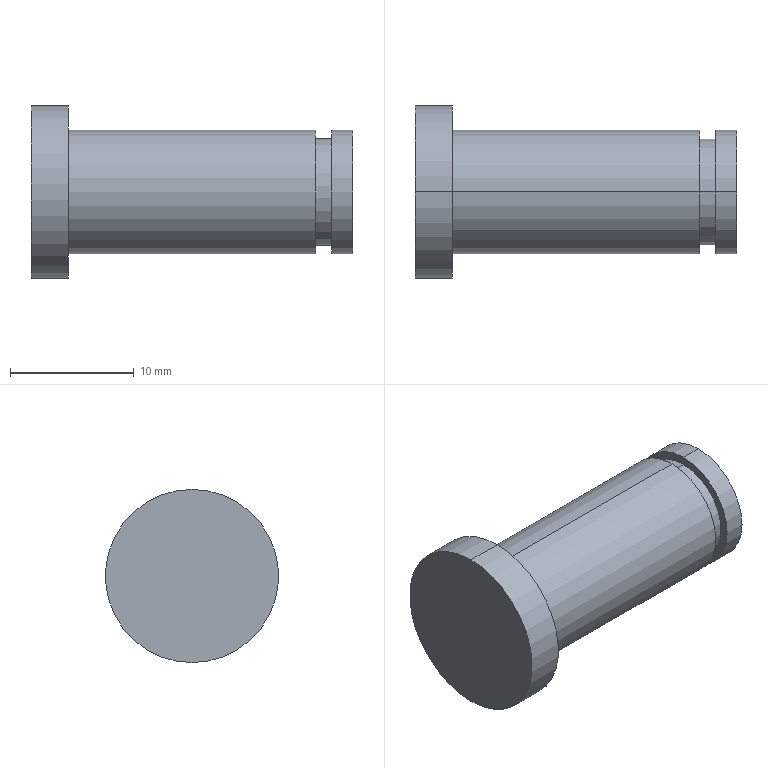Component | SolidWorks | OT-0200-012(PinShaft)-1 | 1 solid | 13 faces | box 26 x 14 x 14 mm | volume 2242 mm3 | cylinder 8 | plane 5 | commonest cylinder face diameters 10 x4 8.6 x2 14 x2 | material Plain Carbon Steel
build123d program:
from build123d import *


with BuildPart() as part:
    # Sketch1 → Revolve1 (revolve)
    with BuildSketch(Plane(origin=(0, 0, 0), x_dir=(1, 0, 0), z_dir=(0, 1, 0))):
        Polygon((0, 7), (0, 0), (26, 0), (26, 5), (24.3, 5), (24.3, 4.3), (23, 4.3), (23, 5), (3, 5), (3, 7), align=None)
    revolve(axis=Axis((26, 0, 0), (-1, 0, 0)))


solid = part.part

# Placed as in the assembly
solid = solid.moved(Location((187, 104.973, -26.996), (0, 0, 0)))
STEP:
#1=CARTESIAN_POINT('',(8.319,4.133,-1.26));
#2=VERTEX_POINT('',#1);
#3=CARTESIAN_POINT('',(8.319,4.133,-0.866));
#4=VERTEX_POINT('',#3);
#5=CARTESIAN_POINT('',(8.319,4.133,-1.063));
#6=DIRECTION('',(1.,0.,0.));
#7=DIRECTION('',(0.,0.,-1.));
#8=AXIS2_PLACEMENT_3D('',#5,#6,#7);
#9=CIRCLE('',#8,0.1969);
#10=EDGE_CURVE('',#2,#4,#9,.T.);
#11=ORIENTED_EDGE('',*,*,#10,.T.);
#12=CARTESIAN_POINT('',(8.386,4.133,-0.866));
#13=VERTEX_POINT('',#12);
#14=CARTESIAN_POINT('',(8.386,4.133,-0.866));
#15=DIRECTION('',(1.,0.,0.));
#16=VECTOR('',#15,39.37);
#17=LINE('',#14,#16);
#18=EDGE_CURVE('',#4,#13,#17,.T.);
#19=ORIENTED_EDGE('',*,*,#18,.T.);
#20=CARTESIAN_POINT('',(8.386,4.133,-1.26));
#21=VERTEX_POINT('',#20);
#22=CARTESIAN_POINT('',(8.386,4.133,-1.063));
#23=DIRECTION('',(1.,0.,0.));
#24=DIRECTION('',(0.,0.,-1.));
#25=AXIS2_PLACEMENT_3D('',#22,#23,#24);
#26=CIRCLE('',#25,0.1969);
#27=EDGE_CURVE('',#21,#13,#26,.T.);
#28=ORIENTED_EDGE('',*,*,#27,.F.);
#29=CARTESIAN_POINT('',(8.386,4.133,-1.26));
#30=DIRECTION('',(1.,0.,0.));
#31=VECTOR('',#30,39.37);
#32=LINE('',#29,#31);
#33=EDGE_CURVE('',#2,#21,#32,.T.);
#34=ORIENTED_EDGE('',*,*,#33,.F.);
#35=EDGE_LOOP('',(#11,#19,#28,#34));
#36=FACE_OUTER_BOUND('',#35,.T.);
#37=CARTESIAN_POINT('',(8.386,4.133,-1.063));
#38=DIRECTION('',(1.,0.,0.));
#39=DIRECTION('',(0.,0.,-1.));
#40=AXIS2_PLACEMENT_3D('',#37,#38,#39);
#41=CYLINDRICAL_SURFACE('',#40,0.1969);
#42=ADVANCED_FACE('',(#36),#41,.T.);
#43=CARTESIAN_POINT('',(8.268,4.133,-1.232));
#44=VERTEX_POINT('',#43);
#45=CARTESIAN_POINT('',(8.268,4.133,-0.8935));
#46=VERTEX_POINT('',#45);
#47=CARTESIAN_POINT('',(8.268,4.133,-1.063));
#48=DIRECTION('',(1.,0.,0.));
#49=DIRECTION('',(0.,0.,-1.));
#50=AXIS2_PLACEMENT_3D('',#47,#48,#49);
#51=CIRCLE('',#50,0.1693);
#52=EDGE_CURVE('',#44,#46,#51,.T.);
#53=ORIENTED_EDGE('',*,*,#52,.T.);
#54=CARTESIAN_POINT('',(8.319,4.133,-0.8935));
#55=VERTEX_POINT('',#54);
#56=CARTESIAN_POINT('',(8.386,4.133,-0.8935));
#57=DIRECTION('',(1.,0.,0.));
#58=VECTOR('',#57,39.37);
#59=LINE('',#56,#58);
#60=EDGE_CURVE('',#46,#55,#59,.T.);
#61=ORIENTED_EDGE('',*,*,#60,.T.);
#62=CARTESIAN_POINT('',(8.319,4.133,-1.232));
#63=VERTEX_POINT('',#62);
#64=CARTESIAN_POINT('',(8.319,4.133,-1.063));
#65=DIRECTION('',(1.,0.,0.));
#66=DIRECTION('',(0.,0.,-1.));
#67=AXIS2_PLACEMENT_3D('',#64,#65,#66);
#68=CIRCLE('',#67,0.1693);
#69=EDGE_CURVE('',#63,#55,#68,.T.);
#70=ORIENTED_EDGE('',*,*,#69,.F.);
#71=CARTESIAN_POINT('',(8.386,4.133,-1.232));
#72=DIRECTION('',(1.,0.,0.));
#73=VECTOR('',#72,39.37);
#74=LINE('',#71,#73);
#75=EDGE_CURVE('',#44,#63,#74,.T.);
#76=ORIENTED_EDGE('',*,*,#75,.F.);
#77=EDGE_LOOP('',(#53,#61,#70,#76));
#78=FACE_OUTER_BOUND('',#77,.T.);
#79=CARTESIAN_POINT('',(8.386,4.133,-1.063));
#80=DIRECTION('',(1.,0.,0.));
#81=DIRECTION('',(0.,0.,-1.));
#82=AXIS2_PLACEMENT_3D('',#79,#80,#81);
#83=CYLINDRICAL_SURFACE('',#82,0.1693);
#84=ADVANCED_FACE('',(#78),#83,.T.);
#85=CARTESIAN_POINT('',(7.48,4.133,-1.26));
#86=VERTEX_POINT('',#85);
#87=CARTESIAN_POINT('',(7.48,4.133,-0.866));
#88=VERTEX_POINT('',#87);
#89=CARTESIAN_POINT('',(7.48,4.133,-1.063));
#90=DIRECTION('',(1.,0.,0.));
#91=DIRECTION('',(0.,0.,-1.));
#92=AXIS2_PLACEMENT_3D('',#89,#90,#91);
#93=CIRCLE('',#92,0.1969);
#94=EDGE_CURVE('',#86,#88,#93,.T.);
#95=ORIENTED_EDGE('',*,*,#94,.T.);
#96=CARTESIAN_POINT('',(8.268,4.133,-0.866));
#97=VERTEX_POINT('',#96);
#98=CARTESIAN_POINT('',(8.386,4.133,-0.866));
#99=DIRECTION('',(1.,0.,0.));
#100=VECTOR('',#99,39.37);
#101=LINE('',#98,#100);
#102=EDGE_CURVE('',#88,#97,#101,.T.);
#103=ORIENTED_EDGE('',*,*,#102,.T.);
#104=CARTESIAN_POINT('',(8.268,4.133,-1.26));
#105=VERTEX_POINT('',#104);
#106=CARTESIAN_POINT('',(8.268,4.133,-1.063));
#107=DIRECTION('',(1.,0.,0.));
#108=DIRECTION('',(0.,0.,-1.));
#109=AXIS2_PLACEMENT_3D('',#106,#107,#108);
#110=CIRCLE('',#109,0.1969);
#111=EDGE_CURVE('',#105,#97,#110,.T.);
#112=ORIENTED_EDGE('',*,*,#111,.F.);
#113=CARTESIAN_POINT('',(8.386,4.133,-1.26));
#114=DIRECTION('',(1.,0.,0.));
#115=VECTOR('',#114,39.37);
#116=LINE('',#113,#115);
#117=EDGE_CURVE('',#86,#105,#116,.T.);
#118=ORIENTED_EDGE('',*,*,#117,.F.);
#119=EDGE_LOOP('',(#95,#103,#112,#118));
#120=FACE_OUTER_BOUND('',#119,.T.);
#121=CARTESIAN_POINT('',(8.386,4.133,-1.063));
#122=DIRECTION('',(1.,0.,0.));
#123=DIRECTION('',(0.,0.,-1.));
#124=AXIS2_PLACEMENT_3D('',#121,#122,#123);
#125=CYLINDRICAL_SURFACE('',#124,0.1969);
#126=ADVANCED_FACE('',(#120),#125,.T.);
#127=CARTESIAN_POINT('',(7.362,4.133,-1.338));
#128=VERTEX_POINT('',#127);
#129=CARTESIAN_POINT('',(7.362,4.133,-0.7872));
#130=VERTEX_POINT('',#129);
#131=CARTESIAN_POINT('',(7.362,4.133,-1.063));
#132=DIRECTION('',(1.,0.,0.));
#133=DIRECTION('',(0.,0.,-1.));
#134=AXIS2_PLACEMENT_3D('',#131,#132,#133);
#135=CIRCLE('',#134,0.2756);
#136=EDGE_CURVE('',#128,#130,#135,.T.);
#137=ORIENTED_EDGE('',*,*,#136,.T.);
#138=CARTESIAN_POINT('',(7.48,4.133,-0.7872));
#139=VERTEX_POINT('',#138);
#140=CARTESIAN_POINT('',(8.386,4.133,-0.7872));
#141=DIRECTION('',(1.,0.,0.));
#142=VECTOR('',#141,39.37);
#143=LINE('',#140,#142);
#144=EDGE_CURVE('',#130,#139,#143,.T.);
#145=ORIENTED_EDGE('',*,*,#144,.T.);
#146=CARTESIAN_POINT('',(7.48,4.133,-1.338));
#147=VERTEX_POINT('',#146);
#148=CARTESIAN_POINT('',(7.48,4.133,-1.063));
#149=DIRECTION('',(1.,0.,0.));
#150=DIRECTION('',(0.,0.,-1.));
#151=AXIS2_PLACEMENT_3D('',#148,#149,#150);
#152=CIRCLE('',#151,0.2756);
#153=EDGE_CURVE('',#147,#139,#152,.T.);
#154=ORIENTED_EDGE('',*,*,#153,.F.);
#155=CARTESIAN_POINT('',(8.386,4.133,-1.338));
#156=DIRECTION('',(1.,0.,0.));
#157=VECTOR('',#156,39.37);
#158=LINE('',#155,#157);
#159=EDGE_CURVE('',#128,#147,#158,.T.);
#160=ORIENTED_EDGE('',*,*,#159,.F.);
#161=EDGE_LOOP('',(#137,#145,#154,#160));
#162=FACE_OUTER_BOUND('',#161,.T.);
#163=CARTESIAN_POINT('',(8.386,4.133,-1.063));
#164=DIRECTION('',(1.,0.,0.));
#165=DIRECTION('',(0.,0.,-1.));
#166=AXIS2_PLACEMENT_3D('',#163,#164,#165);
#167=CYLINDRICAL_SURFACE('',#166,0.2756);
#168=ADVANCED_FACE('',(#162),#167,.T.);
#169=ORIENTED_EDGE('',*,*,#144,.F.);
#170=CARTESIAN_POINT('',(7.362,4.133,-1.063));
#171=DIRECTION('',(1.,0.,0.));
#172=DIRECTION('',(0.,0.,-1.));
#173=AXIS2_PLACEMENT_3D('',#170,#171,#172);
#174=CIRCLE('',#173,0.2756);
#175=EDGE_CURVE('',#130,#128,#174,.T.);
#176=ORIENTED_EDGE('',*,*,#175,.T.);
#177=ORIENTED_EDGE('',*,*,#159,.T.);
#178=CARTESIAN_POINT('',(7.48,4.133,-1.063));
#179=DIRECTION('',(1.,0.,0.));
#180=DIRECTION('',(0.,0.,-1.));
#181=AXIS2_PLACEMENT_3D('',#178,#179,#180);
#182=CIRCLE('',#181,0.2756);
#183=EDGE_CURVE('',#139,#147,#182,.T.);
#184=ORIENTED_EDGE('',*,*,#183,.F.);
#185=EDGE_LOOP('',(#169,#176,#177,#184));
#186=FACE_OUTER_BOUND('',#185,.T.);
#187=CARTESIAN_POINT('',(8.386,4.133,-1.063));
#188=DIRECTION('',(1.,0.,0.));
#189=DIRECTION('',(0.,0.,-1.));
#190=AXIS2_PLACEMENT_3D('',#187,#188,#189);
#191=CYLINDRICAL_SURFACE('',#190,0.2756);
#192=ADVANCED_FACE('',(#186),#191,.T.);
#193=ORIENTED_EDGE('',*,*,#153,.T.);
#194=ORIENTED_EDGE('',*,*,#183,.T.);
#195=EDGE_LOOP('',(#193,#194));
#196=FACE_OUTER_BOUND('',#195,.T.);
#197=ORIENTED_EDGE('',*,*,#94,.F.);
#198=CARTESIAN_POINT('',(7.48,4.133,-1.063));
#199=DIRECTION('',(1.,0.,0.));
#200=DIRECTION('',(0.,0.,-1.));
#201=AXIS2_PLACEMENT_3D('',#198,#199,#200);
#202=CIRCLE('',#201,0.1969);
#203=EDGE_CURVE('',#88,#86,#202,.T.);
#204=ORIENTED_EDGE('',*,*,#203,.F.);
#205=EDGE_LOOP('',(#197,#204));
#206=FACE_BOUND('',#205,.T.);
#207=CARTESIAN_POINT('',(7.48,4.133,-1.338));
#208=DIRECTION('',(1.,0.,0.));
#209=DIRECTION('',(0.,0.,-1.));
#210=AXIS2_PLACEMENT_3D('',#207,#208,#209);
#211=PLANE('',#210);
#212=ADVANCED_FACE('',(#196,#206),#211,.T.);
#213=ORIENTED_EDGE('',*,*,#102,.F.);
#214=ORIENTED_EDGE('',*,*,#203,.T.);
#215=ORIENTED_EDGE('',*,*,#117,.T.);
#216=CARTESIAN_POINT('',(8.268,4.133,-1.063));
#217=DIRECTION('',(1.,0.,0.));
#218=DIRECTION('',(0.,0.,-1.));
#219=AXIS2_PLACEMENT_3D('',#216,#217,#218);
#220=CIRCLE('',#219,0.1969);
#221=EDGE_CURVE('',#97,#105,#220,.T.);
#222=ORIENTED_EDGE('',*,*,#221,.F.);
#223=EDGE_LOOP('',(#213,#214,#215,#222));
#224=FACE_OUTER_BOUND('',#223,.T.);
#225=CARTESIAN_POINT('',(8.386,4.133,-1.063));
#226=DIRECTION('',(1.,0.,0.));
#227=DIRECTION('',(0.,0.,-1.));
#228=AXIS2_PLACEMENT_3D('',#225,#226,#227);
#229=CYLINDRICAL_SURFACE('',#228,0.1969);
#230=ADVANCED_FACE('',(#224),#229,.T.);
#231=ORIENTED_EDGE('',*,*,#111,.T.);
#232=ORIENTED_EDGE('',*,*,#221,.T.);
#233=EDGE_LOOP('',(#231,#232));
#234=FACE_OUTER_BOUND('',#233,.T.);
#235=ORIENTED_EDGE('',*,*,#52,.F.);
#236=CARTESIAN_POINT('',(8.268,4.133,-1.063));
#237=DIRECTION('',(1.,0.,0.));
#238=DIRECTION('',(0.,0.,-1.));
#239=AXIS2_PLACEMENT_3D('',#236,#237,#238);
#240=CIRCLE('',#239,0.1693);
#241=EDGE_CURVE('',#46,#44,#240,.T.);
#242=ORIENTED_EDGE('',*,*,#241,.F.);
#243=EDGE_LOOP('',(#235,#242));
#244=FACE_BOUND('',#243,.T.);
#245=CARTESIAN_POINT('',(8.268,4.133,-1.26));
#246=DIRECTION('',(1.,0.,0.));
#247=DIRECTION('',(0.,0.,-1.));
#248=AXIS2_PLACEMENT_3D('',#245,#246,#247);
#249=PLANE('',#248);
#250=ADVANCED_FACE('',(#234,#244),#249,.T.);
#251=ORIENTED_EDGE('',*,*,#60,.F.);
#252=ORIENTED_EDGE('',*,*,#241,.T.);
#253=ORIENTED_EDGE('',*,*,#75,.T.);
#254=CARTESIAN_POINT('',(8.319,4.133,-1.063));
#255=DIRECTION('',(1.,0.,0.));
#256=DIRECTION('',(0.,0.,-1.));
#257=AXIS2_PLACEMENT_3D('',#254,#255,#256);
#258=CIRCLE('',#257,0.1693);
#259=EDGE_CURVE('',#55,#63,#258,.T.);
#260=ORIENTED_EDGE('',*,*,#259,.F.);
#261=EDGE_LOOP('',(#251,#252,#253,#260));
#262=FACE_OUTER_BOUND('',#261,.T.);
#263=CARTESIAN_POINT('',(8.386,4.133,-1.063));
#264=DIRECTION('',(1.,0.,0.));
#265=DIRECTION('',(0.,0.,-1.));
#266=AXIS2_PLACEMENT_3D('',#263,#264,#265);
#267=CYLINDRICAL_SURFACE('',#266,0.1693);
#268=ADVANCED_FACE('',(#262),#267,.T.);
#269=ORIENTED_EDGE('',*,*,#69,.T.);
#270=ORIENTED_EDGE('',*,*,#259,.T.);
#271=EDGE_LOOP('',(#269,#270));
#272=FACE_BOUND('',#271,.T.);
#273=ORIENTED_EDGE('',*,*,#10,.F.);
#274=CARTESIAN_POINT('',(8.319,4.133,-1.063));
#275=DIRECTION('',(1.,0.,0.));
#276=DIRECTION('',(0.,0.,-1.));
#277=AXIS2_PLACEMENT_3D('',#274,#275,#276);
#278=CIRCLE('',#277,0.1969);
#279=EDGE_CURVE('',#4,#2,#278,.T.);
#280=ORIENTED_EDGE('',*,*,#279,.F.);
#281=EDGE_LOOP('',(#273,#280));
#282=FACE_OUTER_BOUND('',#281,.T.);
#283=CARTESIAN_POINT('',(8.319,4.133,-1.232));
#284=DIRECTION('',(-1.,0.,-0.));
#285=DIRECTION('',(-0.,0.,1.));
#286=AXIS2_PLACEMENT_3D('',#283,#284,#285);
#287=PLANE('',#286);
#288=ADVANCED_FACE('',(#272,#282),#287,.T.);
#289=ORIENTED_EDGE('',*,*,#18,.F.);
#290=ORIENTED_EDGE('',*,*,#279,.T.);
#291=ORIENTED_EDGE('',*,*,#33,.T.);
#292=CARTESIAN_POINT('',(8.386,4.133,-1.063));
#293=DIRECTION('',(1.,0.,0.));
#294=DIRECTION('',(0.,0.,-1.));
#295=AXIS2_PLACEMENT_3D('',#292,#293,#294);
#296=CIRCLE('',#295,0.1969);
#297=EDGE_CURVE('',#13,#21,#296,.T.);
#298=ORIENTED_EDGE('',*,*,#297,.F.);
#299=EDGE_LOOP('',(#289,#290,#291,#298));
#300=FACE_OUTER_BOUND('',#299,.T.);
#301=CARTESIAN_POINT('',(8.386,4.133,-1.063));
#302=DIRECTION('',(1.,0.,0.));
#303=DIRECTION('',(0.,0.,-1.));
#304=AXIS2_PLACEMENT_3D('',#301,#302,#303);
#305=CYLINDRICAL_SURFACE('',#304,0.1969);
#306=ADVANCED_FACE('',(#300),#305,.T.);
#307=ORIENTED_EDGE('',*,*,#27,.T.);
#308=ORIENTED_EDGE('',*,*,#297,.T.);
#309=EDGE_LOOP('',(#307,#308));
#310=FACE_OUTER_BOUND('',#309,.T.);
#311=CARTESIAN_POINT('',(8.386,4.133,-1.26));
#312=DIRECTION('',(1.,0.,0.));
#313=DIRECTION('',(0.,0.,-1.));
#314=AXIS2_PLACEMENT_3D('',#311,#312,#313);
#315=PLANE('',#314);
#316=ADVANCED_FACE('',(#310),#315,.T.);
#317=ORIENTED_EDGE('',*,*,#136,.F.);
#318=ORIENTED_EDGE('',*,*,#175,.F.);
#319=EDGE_LOOP('',(#317,#318));
#320=FACE_OUTER_BOUND('',#319,.T.);
#321=CARTESIAN_POINT('',(7.362,4.133,-1.338));
#322=DIRECTION('',(-1.,0.,-0.));
#323=DIRECTION('',(-0.,0.,1.));
#324=AXIS2_PLACEMENT_3D('',#321,#322,#323);
#325=PLANE('',#324);
#326=ADVANCED_FACE('',(#320),#325,.T.);
#327=CLOSED_SHELL('',(#42,#84,#126,#168,#192,#212,#230,#250,#268,#288,#306,#316,#326));
#328=MANIFOLD_SOLID_BREP('',#327);
#329=CARTESIAN_POINT('',(0.,0.,0.));
#330=DIRECTION('',(0.,0.,1.));
#331=DIRECTION('',(1.,0.,0.));
#332=AXIS2_PLACEMENT_3D('',#329,#330,#331);
#333=(LENGTH_UNIT()NAMED_UNIT(*)SI_UNIT($,.METRE.));
#334=LENGTH_MEASURE_WITH_UNIT(LENGTH_MEASURE(0.0254),#333);
#335=DIMENSIONAL_EXPONENTS(1.,0.,0.,0.,0.,0.,0.);
#336=(CONVERSION_BASED_UNIT('',#334)LENGTH_UNIT()NAMED_UNIT(#335));
#337=UNCERTAINTY_MEASURE_WITH_UNIT(LENGTH_MEASURE(0.00001),#336,'','');
#338=(NAMED_UNIT(*)PLANE_ANGLE_UNIT()SI_UNIT($,.RADIAN.));
#339=(NAMED_UNIT(*)SI_UNIT($,.STERADIAN.)SOLID_ANGLE_UNIT());
#340=(GEOMETRIC_REPRESENTATION_CONTEXT(3)GLOBAL_UNCERTAINTY_ASSIGNED_CONTEXT((#337))GLOBAL_UNIT_ASSIGNED_CONTEXT((#336,#338,#339))REPRESENTATION_CONTEXT('',''));
#341=ADVANCED_BREP_SHAPE_REPRESENTATION('',(#328,#332),#340);
#342=COLOUR_RGB('',0.7922,0.8196,0.9333);
#343=FILL_AREA_STYLE_COLOUR('',#342);
#344=FILL_AREA_STYLE('',(#343));
#345=SURFACE_STYLE_FILL_AREA(#344);
#346=SURFACE_SIDE_STYLE('',(#345));
#347=SURFACE_STYLE_USAGE(.BOTH.,#346);
#348=PRESENTATION_STYLE_ASSIGNMENT((#347));
#349=STYLED_ITEM('',(#348),#328);
#350=(LENGTH_UNIT()NAMED_UNIT(*)SI_UNIT($,.METRE.));
#351=LENGTH_MEASURE_WITH_UNIT(LENGTH_MEASURE(0.0254),#350);
#352=DIMENSIONAL_EXPONENTS(1.,0.,0.,0.,0.,0.,0.);
#353=(CONVERSION_BASED_UNIT('',#351)LENGTH_UNIT()NAMED_UNIT(#352));
#354=UNCERTAINTY_MEASURE_WITH_UNIT(LENGTH_MEASURE(0.00001),#353,'','');
#355=(NAMED_UNIT(*)PLANE_ANGLE_UNIT()SI_UNIT($,.RADIAN.));
#356=(NAMED_UNIT(*)SI_UNIT($,.STERADIAN.)SOLID_ANGLE_UNIT());
#357=(GEOMETRIC_REPRESENTATION_CONTEXT(3)GLOBAL_UNCERTAINTY_ASSIGNED_CONTEXT((#354))GLOBAL_UNIT_ASSIGNED_CONTEXT((#353,#355,#356))REPRESENTATION_CONTEXT('',''));
#358=MECHANICAL_DESIGN_GEOMETRIC_PRESENTATION_REPRESENTATION('',(#349),#357);
#359=PRESENTATION_LAYER_ASSIGNMENT('','',(#349));